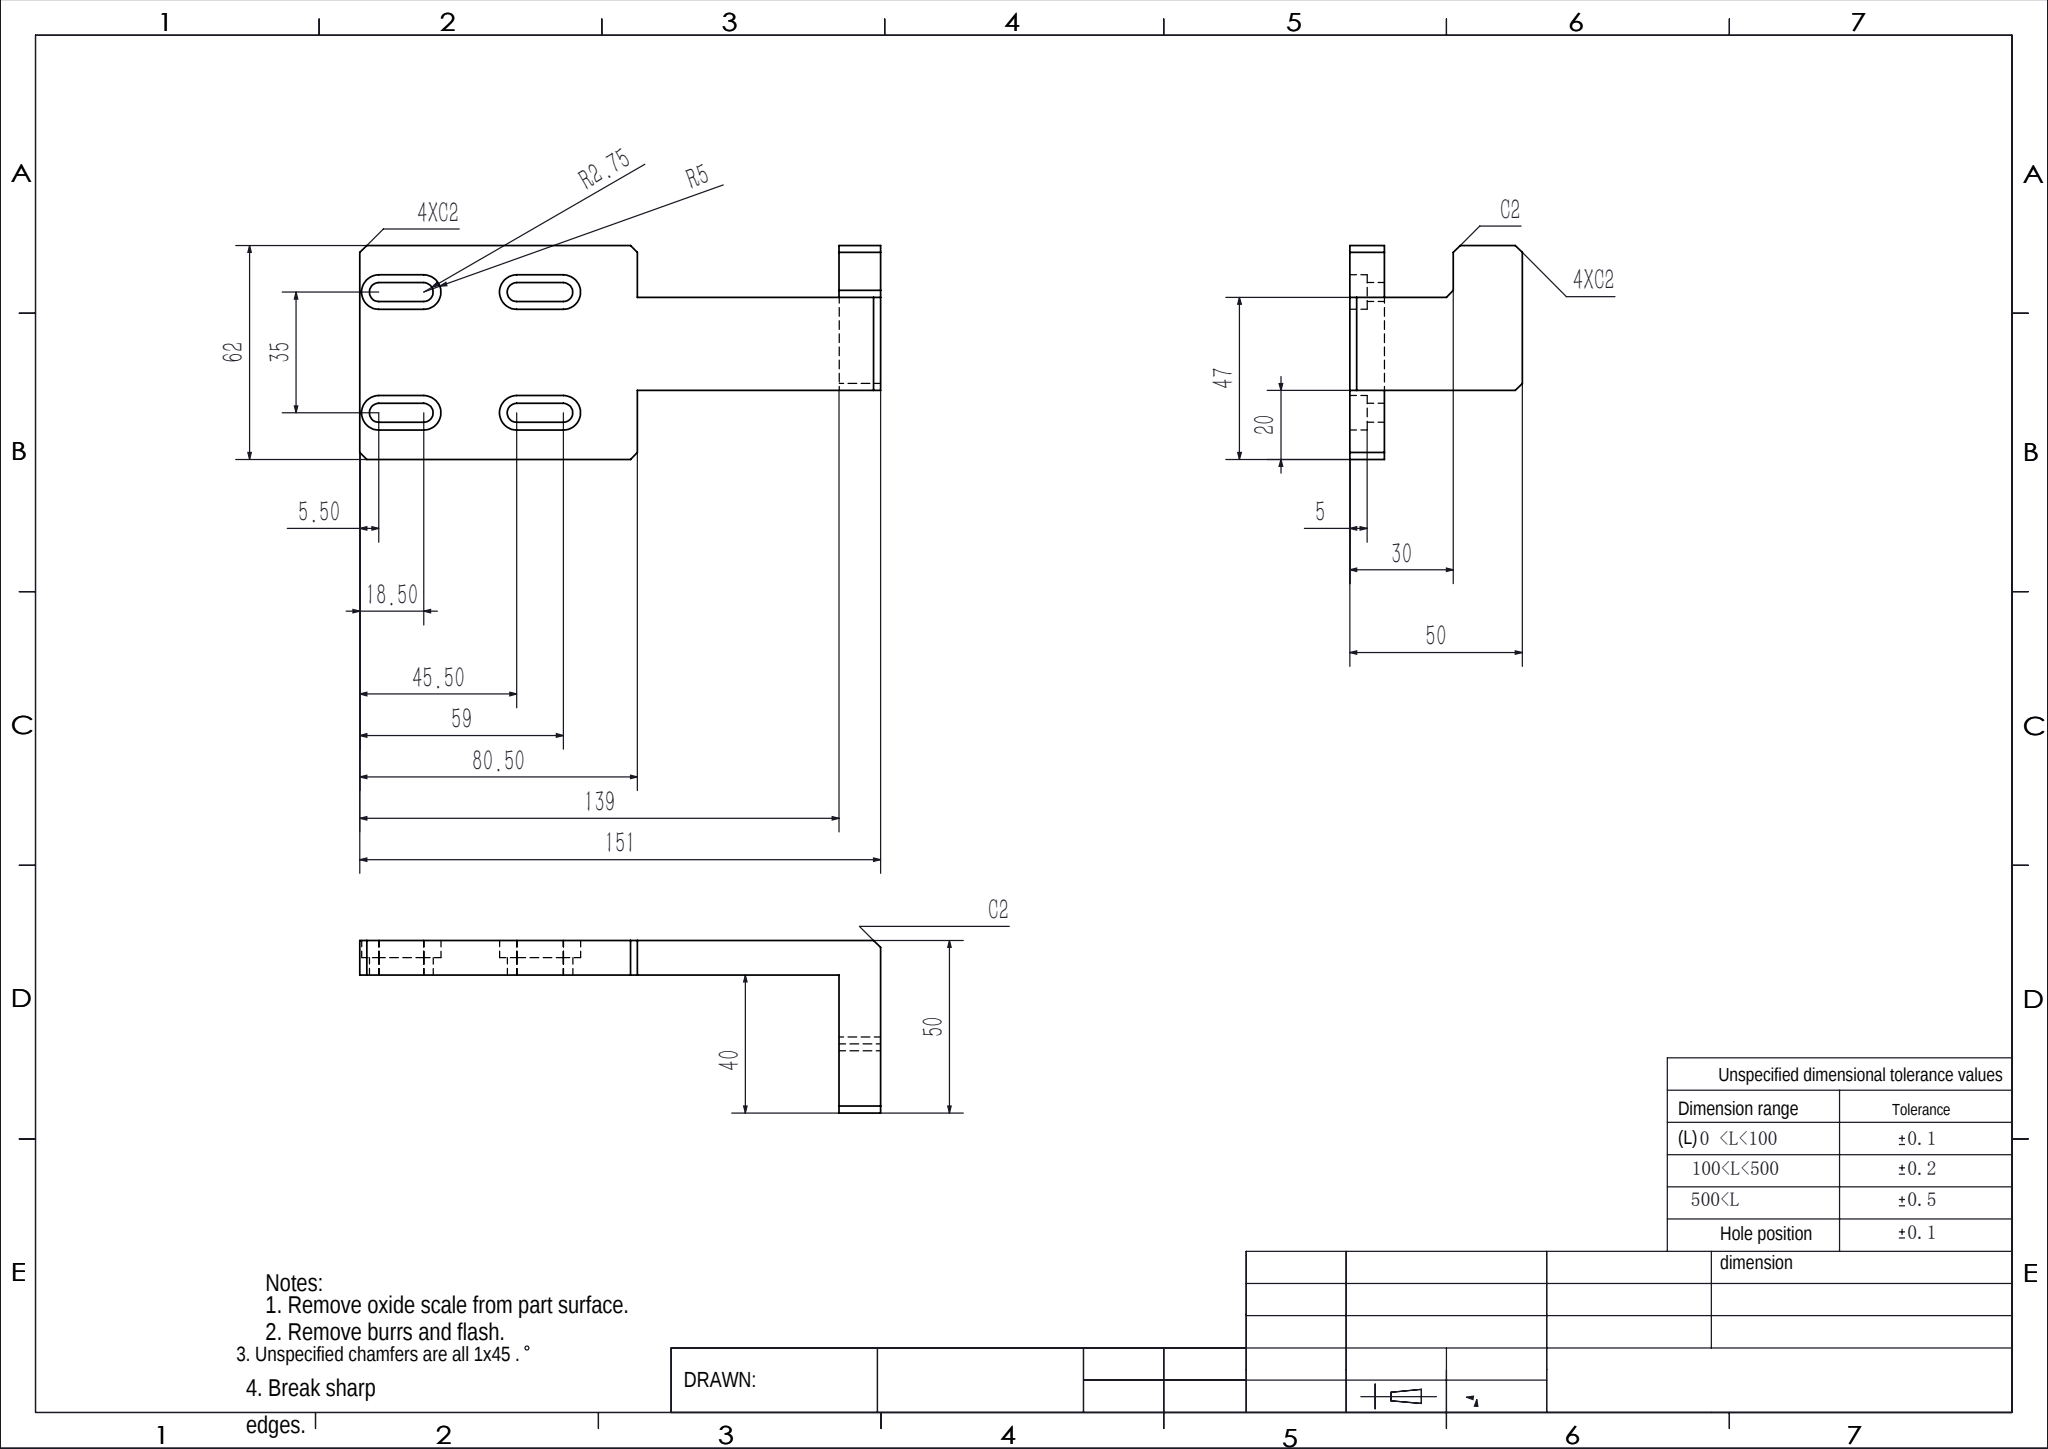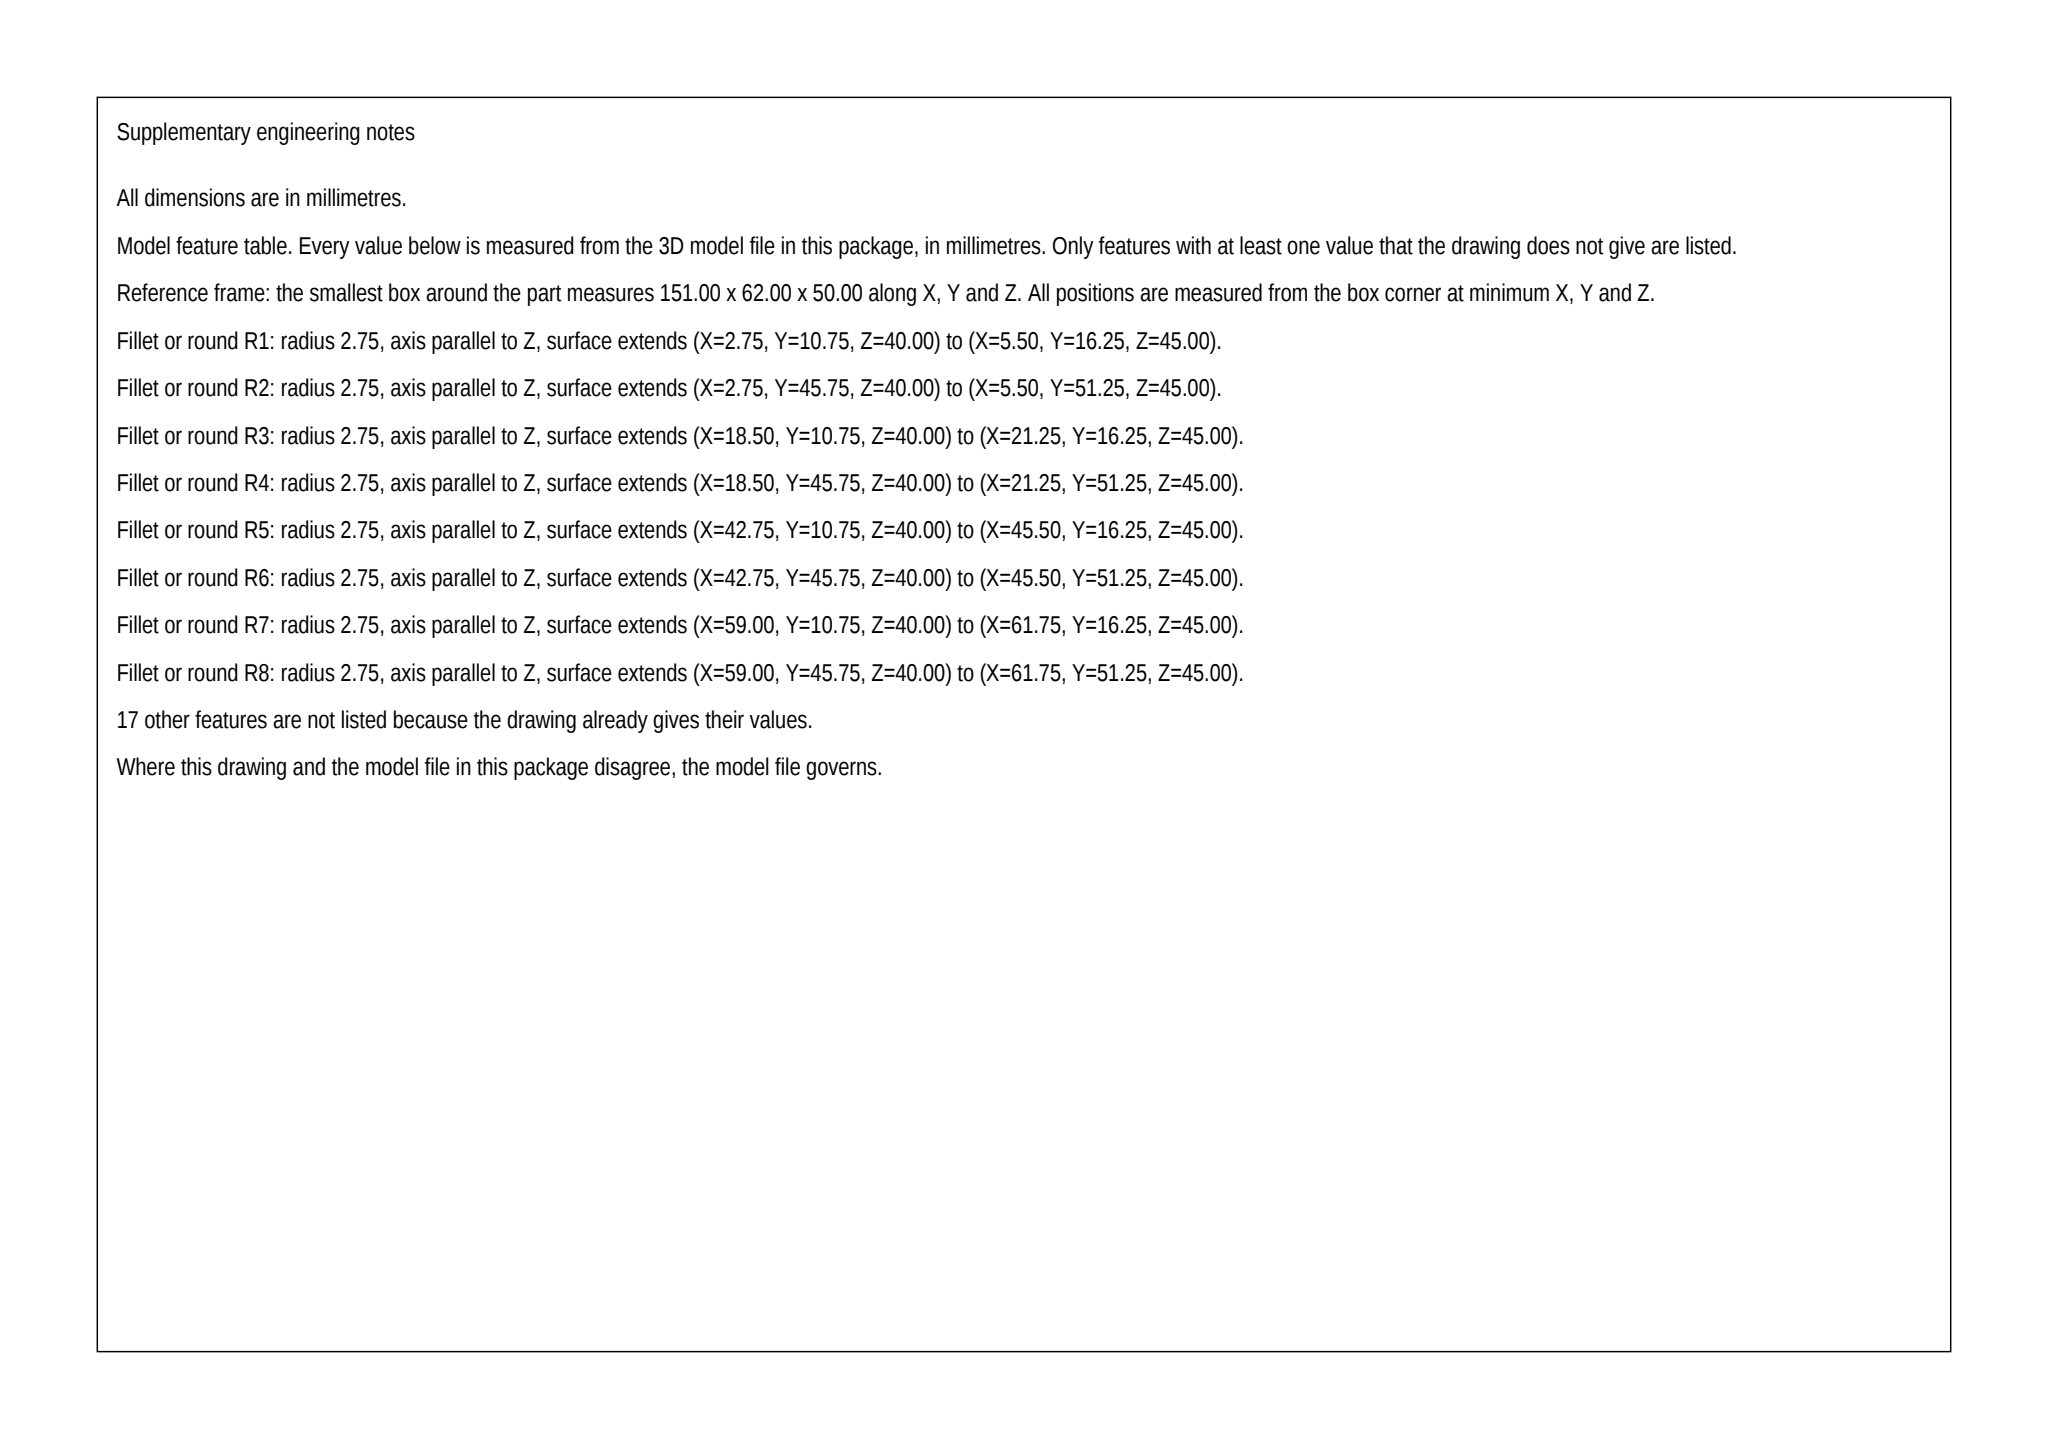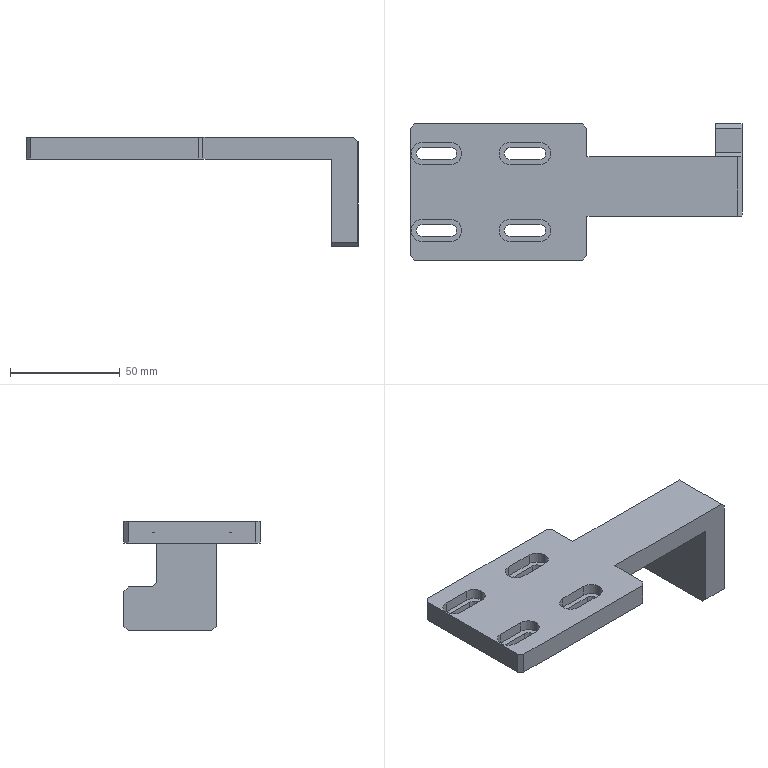Part | SolidWorks | mm | 1 solid | 67 faces | box 151 x 62 x 50 mm | volume 79170 mm3 | plane 43 | cylinder 24 | commonest cylinder face diameters 10 x12 5.5 x12
Drawing notes:
SHARP CORNERS AT X80.5 STEP AND X139/151 LEG - NO FILLETS | from the solid: fillet_radii list empty; x planes 80.5, 139.0, 151.0
PLATE THK 10 (Z40-Z50); NOTE 'PLATE THK 5' VOID | from the solid: Planes z=40 (x0-139,y0-62) and z=50 (x0-149,y0-62) bound plate: 10 thk
4X SLOT R5 CBORE DP 5 FROM TOP FACE; 5.5 WIDE SLOT THRU | from the solid: Ø10 arcs z45-50, Ø5.5 arcs z40-45 at x5.5/18.5/45.5/59, y13.5/48.5
3. UNSPECIFIED CHAMFERS 1X45°. BLUNT SHARP EDGES | from the solid: Inclined planes at 45/45/90 deg to axes, 2x2 legs (C2) confirm 45 deg chamfers
build123d program:
from build123d import *

# Parameters (mm, degrees)
SKETCH1_W           = 156
SKETCH1_H           = 62
BOSS_EXTRUDE1_DEPTH = 10
SKETCH2_W           = 12
SKETCH2_H           = 62
BOSS_EXTRUDE2_DEPTH = 40
CUT_EXTRUDE1_START  = -50
SKETCH3_W           = 12
SKETCH3_H           = 20
CUT_EXTRUDE1_DEPTH  = 50
SKETCH4_W           = 58.5
SKETCH4_H           = 20
CUT_EXTRUDE2_DEPTH  = 10
CHAMFER1_SIZE       = 2
SKETCH5_W           = 30
SKETCH5_H           = 15
CUT_EXTRUDE3_DEPTH  = 70.5
CHAMFER3_SIZE       = 2
CUT_EXTRUDE4_DEPTH  = 10
SKETCH7_W           = 5
SKETCH7_H           = 62
CUT_EXTRUDE5_DEPTH  = 10
CHAMFER5_SIZE       = 2
CHAMFER6_SIZE       = 2
CHAMFER7_SIZE       = 2
CHAMFER8_SIZE       = 2
CUT_EXTRUDE6_DEPTH  = 5


with BuildPart() as part:
    # Sketch1 → Boss-Extrude1 (new body)
    with BuildSketch(Plane.XY):
        Rectangle(SKETCH1_W, SKETCH1_H)
    extrude(amount=BOSS_EXTRUDE1_DEPTH)

    # Sketch2 → Boss-Extrude2 (add)
    with BuildSketch(Plane(origin=(0, 0, 0), x_dir=(-1, 0, 0), z_dir=(0, 0, -1))):
        with Locations((-72, 0)):
            Rectangle(SKETCH2_W, SKETCH2_H)
    extrude(amount=BOSS_EXTRUDE2_DEPTH)

    # Sketch3 → Cut-Extrude1 (cut)
    with BuildSketch(Plane(origin=(0, 0, -40), x_dir=(-1, 0, 0), z_dir=(0, 0, -1)).offset(CUT_EXTRUDE1_START)):
        with Locations((-72, -21)):
            Rectangle(SKETCH3_W, SKETCH3_H)
    extrude(amount=CUT_EXTRUDE1_DEPTH, mode=Mode.SUBTRACT)

    # Sketch4 → Cut-Extrude2 (cut)
    with BuildSketch(Plane.XY.offset(10)):
        with Locations((36.75, -21)):
            Rectangle(SKETCH4_W, SKETCH4_H)
    extrude(amount=-CUT_EXTRUDE2_DEPTH, mode=Mode.SUBTRACT)

    # Chamfer1
    chamfer1_edges = [part.edges().sort_by_distance(p)[0] for p in [
        (72, 31, -40),
        (72, -11, -40),
    ]]
    chamfer(chamfer1_edges, length=CHAMFER1_SIZE)

    # Sketch5 → Cut-Extrude3 (cut)
    with BuildSketch(Plane(origin=(78, 0, 0), x_dir=(0, 0, -1), z_dir=(1, 0, 0))):
        with Locations((5, 23.5)):
            Rectangle(SKETCH5_W, SKETCH5_H)
    extrude(amount=-CUT_EXTRUDE3_DEPTH, mode=Mode.SUBTRACT)

    # Chamfer3
    chamfer3_edges = [part.edges().sort_by_distance(p)[0] for p in [
        (7.5, 31, 5),
        (7.5, -31, 5),
    ]]
    chamfer(chamfer3_edges, length=CHAMFER3_SIZE)

    # Sketch6 → Cut-Extrude4 (cut)
    with BuildSketch(Plane.XY.offset(10)):
        with BuildLine():
            Line((-67.5, 14.75), (-54.5, 14.75))
            ThreePointArc((-54.5, 14.75), (-51.75, 17.5), (-54.5, 20.25))
            Line((-54.5, 20.25), (-67.5, 20.25))
            ThreePointArc((-67.5, 20.25), (-70.25, 17.5), (-67.5, 14.75))
        make_face()
        with BuildLine():
            Line((-27.5, -20.25), (-14, -20.25))
            ThreePointArc((-14, -20.25), (-11.25, -17.5), (-14, -14.75))
            Line((-14, -14.75), (-27.5, -14.75))
            ThreePointArc((-27.5, -14.75), (-30.25, -17.5), (-27.5, -20.25))
        make_face()
        with BuildLine():
            Line((-67.5, -20.25), (-54.5, -20.25))
            ThreePointArc((-54.5, -20.25), (-51.75, -17.5), (-54.5, -14.75))
            Line((-54.5, -14.75), (-67.5, -14.75))
            ThreePointArc((-67.5, -14.75), (-70.25, -17.5), (-67.5, -20.25))
        make_face()
        with BuildLine():
            Line((-27.5, 14.75), (-14, 14.75))
            ThreePointArc((-14, 14.75), (-11.25, 17.5), (-14, 20.25))
            Line((-14, 20.25), (-27.5, 20.25))
            ThreePointArc((-27.5, 20.25), (-30.25, 17.5), (-27.5, 14.75))
        make_face()
    extrude(amount=-CUT_EXTRUDE4_DEPTH, mode=Mode.SUBTRACT)

    # Sketch7 → Cut-Extrude5 (cut)
    with BuildSketch(Plane.XY.offset(10)):
        with Locations((-75.5, 0)):
            Rectangle(SKETCH7_W, SKETCH7_H)
    extrude(amount=-CUT_EXTRUDE5_DEPTH, mode=Mode.SUBTRACT)

    # Chamfer5
    chamfer5_edges = [part.edges().sort_by_distance(p)[0] for p in [
        (72, 31, -20),
    ]]
    chamfer(chamfer5_edges, length=CHAMFER5_SIZE)

    # Chamfer6
    chamfer6_edges = [part.edges().sort_by_distance(p)[0] for p in [
        (72, 16, -20),
    ]]
    chamfer(chamfer6_edges, length=CHAMFER6_SIZE)

    # Chamfer7
    chamfer7_edges = [part.edges().sort_by_distance(p)[0] for p in [
        (78, 2.5, 10),
    ]]
    chamfer(chamfer7_edges, length=CHAMFER7_SIZE)

    # Chamfer8
    chamfer8_edges = [part.edges().sort_by_distance(p)[0] for p in [
        (-73, -31, 5),
        (-73, 31, 5),
    ]]
    chamfer(chamfer8_edges, length=CHAMFER8_SIZE)

    # Sketch8 → Cut-Extrude6 (cut)
    with BuildSketch(Plane.XY.offset(10)):
        with BuildLine():
            Line((-67.5, 22.5), (-54.5, 22.5))
            ThreePointArc((-54.5, 22.5), (-49.5, 17.5), (-54.5, 12.5))
            Line((-54.5, 12.5), (-67.5, 12.5))
            ThreePointArc((-67.5, 12.5), (-72.5, 17.5), (-67.5, 22.5))
        make_face()
        with BuildLine():
            Line((-27.5, 22.5), (-14, 22.5))
            ThreePointArc((-14, 22.5), (-9, 17.5), (-14, 12.5))
            Line((-14, 12.5), (-27.5, 12.5))
            ThreePointArc((-27.5, 12.5), (-32.5, 17.5), (-27.5, 22.5))
        make_face()
        with BuildLine():
            Line((-27.5, -12.5), (-14, -12.5))
            ThreePointArc((-14, -12.5), (-9, -17.5), (-14, -22.5))
            Line((-14, -22.5), (-27.5, -22.5))
            ThreePointArc((-27.5, -22.5), (-32.5, -17.5), (-27.5, -12.5))
        make_face()
        with BuildLine():
            Line((-67.5, -12.5), (-54.5, -12.5))
            ThreePointArc((-54.5, -12.5), (-49.5, -17.5), (-54.5, -22.5))
            Line((-54.5, -22.5), (-67.5, -22.5))
            ThreePointArc((-67.5, -22.5), (-72.5, -17.5), (-67.5, -12.5))
        make_face()
    extrude(amount=-CUT_EXTRUDE6_DEPTH, mode=Mode.SUBTRACT)


solid = part.part